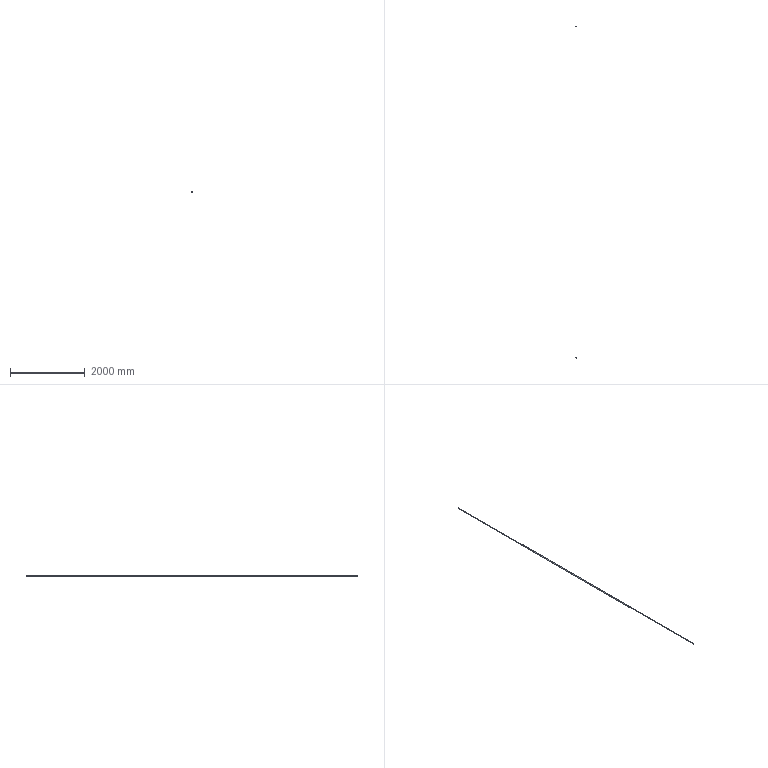Component | NX | 44_6 | 1 solid | 4 faces | volume 1004757 mm3 | cylinder 2 | plane 2 | commonest cylinder face diameters 20 x1 16 x1